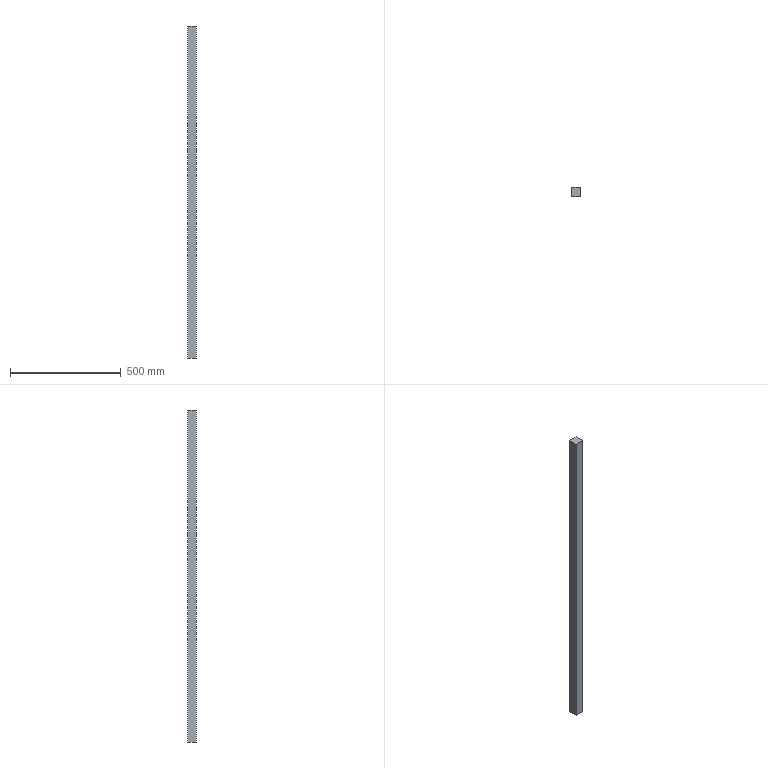Component | SolidWorks | SofaBackrest-1_TieRod-4 | 1 solid | 6 faces | box 40 x 40 x 1500 mm | volume 2400000 mm3 | plane 6
build123d program:
from build123d import *

# Parameters (mm, degrees)
SKETCH1_W           = 40
SKETCH1_H           = 40
BOSS_EXTRUDE1_DEPTH = 1500


with BuildPart() as part:
    # Sketch1 → Boss-Extrude1 (new body)
    with BuildSketch(Plane.XY):
        with Locations((-12.665, -1.306)):
            Rectangle(SKETCH1_W, SKETCH1_H)
    extrude(amount=BOSS_EXTRUDE1_DEPTH)


solid = part.part

# Placed as in the assembly
solid = solid.moved(Location((704.657, 50.526, 830), (0, 0, 0)))
STEP:
#1=COLOUR_RGB('',0.7922,0.8196,0.9333);
#2=FILL_AREA_STYLE_COLOUR('',#1);
#3=FILL_AREA_STYLE('',(#2));
#4=SURFACE_STYLE_FILL_AREA(#3);
#5=SURFACE_SIDE_STYLE('',(#4));
#6=SURFACE_STYLE_USAGE(.BOTH.,#5);
#7=PRESENTATION_STYLE_ASSIGNMENT((#6));
#8=CARTESIAN_POINT('',(26.456,2.725,32.677));
#9=VERTEX_POINT('',#8);
#10=CARTESIAN_POINT('',(26.456,1.15,32.677));
#11=VERTEX_POINT('',#10);
#12=CARTESIAN_POINT('',(26.456,2.725,32.677));
#13=DIRECTION('',(0.,-1.,0.));
#14=VECTOR('',#13,39.37);
#15=LINE('',#12,#14);
#16=EDGE_CURVE('',#9,#11,#15,.T.);
#17=ORIENTED_EDGE('',*,*,#16,.T.);
#18=CARTESIAN_POINT('',(26.456,1.15,91.732));
#19=VERTEX_POINT('',#18);
#20=CARTESIAN_POINT('',(26.456,1.15,91.732));
#21=DIRECTION('',(0.,0.,-1.));
#22=VECTOR('',#21,39.37);
#23=LINE('',#20,#22);
#24=EDGE_CURVE('',#19,#11,#23,.T.);
#25=ORIENTED_EDGE('',*,*,#24,.F.);
#26=CARTESIAN_POINT('',(26.456,2.725,91.732));
#27=VERTEX_POINT('',#26);
#28=CARTESIAN_POINT('',(26.456,2.725,91.732));
#29=DIRECTION('',(0.,-1.,0.));
#30=VECTOR('',#29,39.37);
#31=LINE('',#28,#30);
#32=EDGE_CURVE('',#27,#19,#31,.T.);
#33=ORIENTED_EDGE('',*,*,#32,.F.);
#34=CARTESIAN_POINT('',(26.456,2.725,91.732));
#35=DIRECTION('',(0.,0.,-1.));
#36=VECTOR('',#35,39.37);
#37=LINE('',#34,#36);
#38=EDGE_CURVE('',#27,#9,#37,.T.);
#39=ORIENTED_EDGE('',*,*,#38,.T.);
#40=EDGE_LOOP('',(#17,#25,#33,#39));
#41=FACE_OUTER_BOUND('',#40,.T.);
#42=CARTESIAN_POINT('',(26.456,2.725,91.732));
#43=DIRECTION('',(1.,0.,0.));
#44=DIRECTION('',(-0.,1.,0.));
#45=AXIS2_PLACEMENT_3D('',#42,#43,#44);
#46=PLANE('',#45);
#47=ADVANCED_FACE('',(#41),#46,.F.);
#48=CARTESIAN_POINT('',(28.031,1.15,32.677));
#49=VERTEX_POINT('',#48);
#50=CARTESIAN_POINT('',(26.456,1.15,32.677));
#51=DIRECTION('',(1.,0.,0.));
#52=VECTOR('',#51,39.37);
#53=LINE('',#50,#52);
#54=EDGE_CURVE('',#11,#49,#53,.T.);
#55=ORIENTED_EDGE('',*,*,#54,.T.);
#56=CARTESIAN_POINT('',(28.031,1.15,91.732));
#57=VERTEX_POINT('',#56);
#58=CARTESIAN_POINT('',(28.031,1.15,91.732));
#59=DIRECTION('',(0.,0.,-1.));
#60=VECTOR('',#59,39.37);
#61=LINE('',#58,#60);
#62=EDGE_CURVE('',#57,#49,#61,.T.);
#63=ORIENTED_EDGE('',*,*,#62,.F.);
#64=CARTESIAN_POINT('',(26.456,1.15,91.732));
#65=DIRECTION('',(1.,0.,0.));
#66=VECTOR('',#65,39.37);
#67=LINE('',#64,#66);
#68=EDGE_CURVE('',#19,#57,#67,.T.);
#69=ORIENTED_EDGE('',*,*,#68,.F.);
#70=ORIENTED_EDGE('',*,*,#24,.T.);
#71=EDGE_LOOP('',(#55,#63,#69,#70));
#72=FACE_OUTER_BOUND('',#71,.T.);
#73=CARTESIAN_POINT('',(26.456,1.15,91.732));
#74=DIRECTION('',(0.,1.,0.));
#75=DIRECTION('',(0.,0.,1.));
#76=AXIS2_PLACEMENT_3D('',#73,#74,#75);
#77=PLANE('',#76);
#78=ADVANCED_FACE('',(#72),#77,.F.);
#79=CARTESIAN_POINT('',(28.031,2.725,32.677));
#80=VERTEX_POINT('',#79);
#81=CARTESIAN_POINT('',(28.031,2.725,32.677));
#82=DIRECTION('',(-0.,1.,0.));
#83=VECTOR('',#82,39.37);
#84=LINE('',#81,#83);
#85=EDGE_CURVE('',#49,#80,#84,.T.);
#86=ORIENTED_EDGE('',*,*,#85,.T.);
#87=CARTESIAN_POINT('',(28.031,2.725,91.732));
#88=VERTEX_POINT('',#87);
#89=CARTESIAN_POINT('',(28.031,2.725,91.732));
#90=DIRECTION('',(0.,0.,-1.));
#91=VECTOR('',#90,39.37);
#92=LINE('',#89,#91);
#93=EDGE_CURVE('',#88,#80,#92,.T.);
#94=ORIENTED_EDGE('',*,*,#93,.F.);
#95=CARTESIAN_POINT('',(28.031,2.725,91.732));
#96=DIRECTION('',(-0.,1.,0.));
#97=VECTOR('',#96,39.37);
#98=LINE('',#95,#97);
#99=EDGE_CURVE('',#57,#88,#98,.T.);
#100=ORIENTED_EDGE('',*,*,#99,.F.);
#101=ORIENTED_EDGE('',*,*,#62,.T.);
#102=EDGE_LOOP('',(#86,#94,#100,#101));
#103=FACE_OUTER_BOUND('',#102,.T.);
#104=CARTESIAN_POINT('',(28.031,2.725,91.732));
#105=DIRECTION('',(-1.,-0.,0.));
#106=DIRECTION('',(0.,-1.,0.));
#107=AXIS2_PLACEMENT_3D('',#104,#105,#106);
#108=PLANE('',#107);
#109=ADVANCED_FACE('',(#103),#108,.F.);
#110=CARTESIAN_POINT('',(26.456,2.725,32.677));
#111=DIRECTION('',(-1.,0.,0.));
#112=VECTOR('',#111,39.37);
#113=LINE('',#110,#112);
#114=EDGE_CURVE('',#80,#9,#113,.T.);
#115=ORIENTED_EDGE('',*,*,#114,.T.);
#116=ORIENTED_EDGE('',*,*,#38,.F.);
#117=CARTESIAN_POINT('',(26.456,2.725,91.732));
#118=DIRECTION('',(-1.,0.,0.));
#119=VECTOR('',#118,39.37);
#120=LINE('',#117,#119);
#121=EDGE_CURVE('',#88,#27,#120,.T.);
#122=ORIENTED_EDGE('',*,*,#121,.F.);
#123=ORIENTED_EDGE('',*,*,#93,.T.);
#124=EDGE_LOOP('',(#115,#116,#122,#123));
#125=FACE_OUTER_BOUND('',#124,.T.);
#126=CARTESIAN_POINT('',(26.456,2.725,91.732));
#127=DIRECTION('',(0.,-1.,0.));
#128=DIRECTION('',(0.,0.,-1.));
#129=AXIS2_PLACEMENT_3D('',#126,#127,#128);
#130=PLANE('',#129);
#131=ADVANCED_FACE('',(#125),#130,.F.);
#132=ORIENTED_EDGE('',*,*,#32,.T.);
#133=ORIENTED_EDGE('',*,*,#68,.T.);
#134=ORIENTED_EDGE('',*,*,#99,.T.);
#135=ORIENTED_EDGE('',*,*,#121,.T.);
#136=EDGE_LOOP('',(#132,#133,#134,#135));
#137=FACE_OUTER_BOUND('',#136,.T.);
#138=CARTESIAN_POINT('',(27.742,1.989,91.732));
#139=DIRECTION('',(0.,0.,1.));
#140=DIRECTION('',(1.,0.,0.));
#141=AXIS2_PLACEMENT_3D('',#138,#139,#140);
#142=PLANE('',#141);
#143=ADVANCED_FACE('',(#137),#142,.T.);
#144=ORIENTED_EDGE('',*,*,#16,.F.);
#145=ORIENTED_EDGE('',*,*,#114,.F.);
#146=ORIENTED_EDGE('',*,*,#85,.F.);
#147=ORIENTED_EDGE('',*,*,#54,.F.);
#148=EDGE_LOOP('',(#144,#145,#146,#147));
#149=FACE_OUTER_BOUND('',#148,.T.);
#150=CARTESIAN_POINT('',(27.742,1.989,32.677));
#151=DIRECTION('',(0.,0.,1.));
#152=DIRECTION('',(1.,0.,0.));
#153=AXIS2_PLACEMENT_3D('',#150,#151,#152);
#154=PLANE('',#153);
#155=ADVANCED_FACE('',(#149),#154,.F.);
#156=CLOSED_SHELL('',(#47,#78,#109,#131,#143,#155));
#157=MANIFOLD_SOLID_BREP('',#156);
#158=STYLED_ITEM('',(#7),#157);
#159=PRESENTATION_LAYER_ASSIGNMENT('','',(#158));
#160=(LENGTH_UNIT()NAMED_UNIT(*)SI_UNIT($,.METRE.));
#161=LENGTH_MEASURE_WITH_UNIT(LENGTH_MEASURE(0.0254),#160);
#162=DIMENSIONAL_EXPONENTS(1.,0.,0.,0.,0.,0.,0.);
#163=(CONVERSION_BASED_UNIT('',#161)LENGTH_UNIT()NAMED_UNIT(#162));
#164=UNCERTAINTY_MEASURE_WITH_UNIT(LENGTH_MEASURE(0.00001),#163,'','');
#165=(NAMED_UNIT(*)PLANE_ANGLE_UNIT()SI_UNIT($,.RADIAN.));
#166=(NAMED_UNIT(*)SI_UNIT($,.STERADIAN.)SOLID_ANGLE_UNIT());
#167=(GEOMETRIC_REPRESENTATION_CONTEXT(3)GLOBAL_UNCERTAINTY_ASSIGNED_CONTEXT((#164))GLOBAL_UNIT_ASSIGNED_CONTEXT((#163,#165,#166))REPRESENTATION_CONTEXT('',''));
#168=MECHANICAL_DESIGN_GEOMETRIC_PRESENTATION_REPRESENTATION('',(#158),#167);
#169=CARTESIAN_POINT('',(0.,0.,0.));
#170=DIRECTION('',(0.,0.,1.));
#171=DIRECTION('',(1.,0.,0.));
#172=AXIS2_PLACEMENT_3D('',#169,#170,#171);
#173=(LENGTH_UNIT()NAMED_UNIT(*)SI_UNIT($,.METRE.));
#174=LENGTH_MEASURE_WITH_UNIT(LENGTH_MEASURE(0.0254),#173);
#175=DIMENSIONAL_EXPONENTS(1.,0.,0.,0.,0.,0.,0.);
#176=(CONVERSION_BASED_UNIT('',#174)LENGTH_UNIT()NAMED_UNIT(#175));
#177=UNCERTAINTY_MEASURE_WITH_UNIT(LENGTH_MEASURE(0.00001),#176,'','');
#178=(NAMED_UNIT(*)PLANE_ANGLE_UNIT()SI_UNIT($,.RADIAN.));
#179=(NAMED_UNIT(*)SI_UNIT($,.STERADIAN.)SOLID_ANGLE_UNIT());
#180=(GEOMETRIC_REPRESENTATION_CONTEXT(3)GLOBAL_UNCERTAINTY_ASSIGNED_CONTEXT((#177))GLOBAL_UNIT_ASSIGNED_CONTEXT((#176,#178,#179))REPRESENTATION_CONTEXT('',''));
#181=ADVANCED_BREP_SHAPE_REPRESENTATION('',(#157,#172),#180);